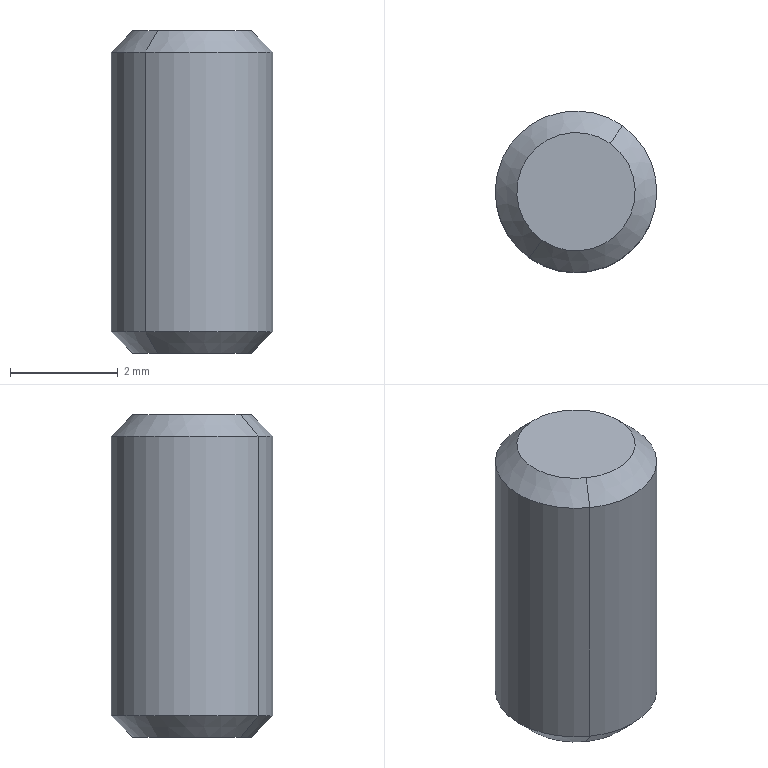Component | SolidWorks | Part28-2 | 1 solid | 8 faces | box 3 x 3 x 6 mm | volume 41 mm3 | cone 4 | cylinder 2 | plane 2 | commonest cylinder face diameters 3 x2
build123d program:
from build123d import *

# Parameters (mm, degrees)
SKETCH1_R           = 1.5
BOSS_EXTRUDE1_DEPTH = 6
CHAMFER1_SIZE       = 0.4


with BuildPart() as part:
    # Sketch1 → Boss-Extrude1 (new body)
    with BuildSketch(Plane.XY):
        Circle(SKETCH1_R)
    extrude(amount=BOSS_EXTRUDE1_DEPTH)

    # Chamfer1
    chamfer1_edges = [part.edges().sort_by_distance(p)[0] for p in [
        (-1.5, 0, 0),
        (-1.5, 0, 6),
    ]]
    chamfer(chamfer1_edges, length=CHAMFER1_SIZE)


solid = part.part

# Placed as in the assembly
solid = solid.moved(Location((65.747, 35.686, -29.938), (0, 0, 0)))
STEP:
#1=COLOUR_RGB('',0.7922,0.8196,0.9333);
#2=FILL_AREA_STYLE_COLOUR('',#1);
#3=FILL_AREA_STYLE('',(#2));
#4=SURFACE_STYLE_FILL_AREA(#3);
#5=SURFACE_SIDE_STYLE('',(#4));
#6=SURFACE_STYLE_USAGE(.BOTH.,#5);
#7=PRESENTATION_STYLE_ASSIGNMENT((#6));
#8=CARTESIAN_POINT('',(2.564,1.37,-0.9424));
#9=VERTEX_POINT('',#8);
#10=CARTESIAN_POINT('',(2.613,1.44,-0.9424));
#11=VERTEX_POINT('',#10);
#12=CARTESIAN_POINT('',(2.588,1.405,-0.9424));
#13=DIRECTION('',(0.,-0.,1.));
#14=DIRECTION('',(-0.5758,-0.8176,0.));
#15=AXIS2_PLACEMENT_3D('',#12,#13,#14);
#16=CIRCLE('',#15,0.04331);
#17=EDGE_CURVE('',#9,#11,#16,.T.);
#18=ORIENTED_EDGE('',*,*,#17,.F.);
#19=CARTESIAN_POINT('',(2.554,1.357,-0.9582));
#20=VERTEX_POINT('',#19);
#21=CARTESIAN_POINT('',(2.564,1.37,-0.9424));
#22=DIRECTION('',(-0.4072,-0.5781,-0.7071));
#23=VECTOR('',#22,39.37);
#24=LINE('',#21,#23);
#25=EDGE_CURVE('',#9,#20,#24,.T.);
#26=ORIENTED_EDGE('',*,*,#25,.T.);
#27=CARTESIAN_POINT('',(2.622,1.453,-0.9582));
#28=VERTEX_POINT('',#27);
#29=CARTESIAN_POINT('',(2.588,1.405,-0.9582));
#30=DIRECTION('',(-0.,0.,-1.));
#31=DIRECTION('',(-0.5758,-0.8176,0.));
#32=AXIS2_PLACEMENT_3D('',#29,#30,#31);
#33=CIRCLE('',#32,0.05906);
#34=EDGE_CURVE('',#28,#20,#33,.T.);
#35=ORIENTED_EDGE('',*,*,#34,.F.);
#36=CARTESIAN_POINT('',(2.613,1.44,-0.9424));
#37=DIRECTION('',(0.4072,0.5781,-0.7071));
#38=VECTOR('',#37,39.37);
#39=LINE('',#36,#38);
#40=EDGE_CURVE('',#11,#28,#39,.T.);
#41=ORIENTED_EDGE('',*,*,#40,.F.);
#42=EDGE_LOOP('',(#18,#26,#35,#41));
#43=FACE_OUTER_BOUND('',#42,.T.);
#44=CARTESIAN_POINT('',(2.588,1.405,-0.9424));
#45=DIRECTION('',(-0.,0.,-1.));
#46=DIRECTION('',(0.5758,0.8176,0.));
#47=AXIS2_PLACEMENT_3D('',#44,#45,#46);
#48=CONICAL_SURFACE('',#47,0.04331,0.7854);
#49=ADVANCED_FACE('',(#43),#48,.T.);
#50=CARTESIAN_POINT('',(2.613,1.44,-1.179));
#51=VERTEX_POINT('',#50);
#52=CARTESIAN_POINT('',(2.564,1.37,-1.179));
#53=VERTEX_POINT('',#52);
#54=CARTESIAN_POINT('',(2.588,1.405,-1.179));
#55=DIRECTION('',(-0.,0.,-1.));
#56=DIRECTION('',(-0.5758,-0.8176,0.));
#57=AXIS2_PLACEMENT_3D('',#54,#55,#56);
#58=CIRCLE('',#57,0.04331);
#59=EDGE_CURVE('',#51,#53,#58,.T.);
#60=ORIENTED_EDGE('',*,*,#59,.F.);
#61=CARTESIAN_POINT('',(2.622,1.453,-1.163));
#62=VERTEX_POINT('',#61);
#63=CARTESIAN_POINT('',(2.622,1.453,-1.163));
#64=DIRECTION('',(0.4072,0.5781,0.7071));
#65=VECTOR('',#64,39.37);
#66=LINE('',#63,#65);
#67=EDGE_CURVE('',#51,#62,#66,.T.);
#68=ORIENTED_EDGE('',*,*,#67,.T.);
#69=CARTESIAN_POINT('',(2.554,1.357,-1.163));
#70=VERTEX_POINT('',#69);
#71=CARTESIAN_POINT('',(2.588,1.405,-1.163));
#72=DIRECTION('',(0.,-0.,1.));
#73=DIRECTION('',(-0.5758,-0.8176,0.));
#74=AXIS2_PLACEMENT_3D('',#71,#72,#73);
#75=CIRCLE('',#74,0.05906);
#76=EDGE_CURVE('',#70,#62,#75,.T.);
#77=ORIENTED_EDGE('',*,*,#76,.F.);
#78=CARTESIAN_POINT('',(2.554,1.357,-1.163));
#79=DIRECTION('',(-0.4072,-0.5781,0.7071));
#80=VECTOR('',#79,39.37);
#81=LINE('',#78,#80);
#82=EDGE_CURVE('',#53,#70,#81,.T.);
#83=ORIENTED_EDGE('',*,*,#82,.F.);
#84=EDGE_LOOP('',(#60,#68,#77,#83));
#85=FACE_OUTER_BOUND('',#84,.T.);
#86=CARTESIAN_POINT('',(2.588,1.405,-1.163));
#87=DIRECTION('',(0.,-0.,1.));
#88=DIRECTION('',(-0.5758,-0.8176,0.));
#89=AXIS2_PLACEMENT_3D('',#86,#87,#88);
#90=CONICAL_SURFACE('',#89,0.05906,0.7854);
#91=ADVANCED_FACE('',(#85),#90,.T.);
#92=ORIENTED_EDGE('',*,*,#34,.T.);
#93=CARTESIAN_POINT('',(2.554,1.357,-0.9424));
#94=DIRECTION('',(-0.,0.,-1.));
#95=VECTOR('',#94,39.37);
#96=LINE('',#93,#95);
#97=EDGE_CURVE('',#20,#70,#96,.T.);
#98=ORIENTED_EDGE('',*,*,#97,.T.);
#99=ORIENTED_EDGE('',*,*,#76,.T.);
#100=CARTESIAN_POINT('',(2.622,1.453,-0.9424));
#101=DIRECTION('',(-0.,0.,-1.));
#102=VECTOR('',#101,39.37);
#103=LINE('',#100,#102);
#104=EDGE_CURVE('',#28,#62,#103,.T.);
#105=ORIENTED_EDGE('',*,*,#104,.F.);
#106=EDGE_LOOP('',(#92,#98,#99,#105));
#107=FACE_OUTER_BOUND('',#106,.T.);
#108=CARTESIAN_POINT('',(2.588,1.405,-0.9424));
#109=DIRECTION('',(-0.,0.,-1.));
#110=DIRECTION('',(0.5758,0.8176,0.));
#111=AXIS2_PLACEMENT_3D('',#108,#109,#110);
#112=CYLINDRICAL_SURFACE('',#111,0.05906);
#113=ADVANCED_FACE('',(#107),#112,.T.);
#114=ORIENTED_EDGE('',*,*,#97,.F.);
#115=CARTESIAN_POINT('',(2.588,1.405,-0.9582));
#116=DIRECTION('',(-0.,0.,-1.));
#117=DIRECTION('',(-0.5758,-0.8176,0.));
#118=AXIS2_PLACEMENT_3D('',#115,#116,#117);
#119=CIRCLE('',#118,0.05906);
#120=EDGE_CURVE('',#20,#28,#119,.T.);
#121=ORIENTED_EDGE('',*,*,#120,.T.);
#122=ORIENTED_EDGE('',*,*,#104,.T.);
#123=CARTESIAN_POINT('',(2.588,1.405,-1.163));
#124=DIRECTION('',(0.,-0.,1.));
#125=DIRECTION('',(-0.5758,-0.8176,0.));
#126=AXIS2_PLACEMENT_3D('',#123,#124,#125);
#127=CIRCLE('',#126,0.05906);
#128=EDGE_CURVE('',#62,#70,#127,.T.);
#129=ORIENTED_EDGE('',*,*,#128,.T.);
#130=EDGE_LOOP('',(#114,#121,#122,#129));
#131=FACE_OUTER_BOUND('',#130,.T.);
#132=CARTESIAN_POINT('',(2.588,1.405,-0.9424));
#133=DIRECTION('',(-0.,0.,-1.));
#134=DIRECTION('',(0.5758,0.8176,0.));
#135=AXIS2_PLACEMENT_3D('',#132,#133,#134);
#136=CYLINDRICAL_SURFACE('',#135,0.05906);
#137=ADVANCED_FACE('',(#131),#136,.T.);
#138=CARTESIAN_POINT('',(2.588,1.405,-0.9424));
#139=DIRECTION('',(0.,-0.,1.));
#140=DIRECTION('',(-0.5758,-0.8176,0.));
#141=AXIS2_PLACEMENT_3D('',#138,#139,#140);
#142=CIRCLE('',#141,0.04331);
#143=EDGE_CURVE('',#11,#9,#142,.T.);
#144=ORIENTED_EDGE('',*,*,#143,.T.);
#145=ORIENTED_EDGE('',*,*,#17,.T.);
#146=EDGE_LOOP('',(#144,#145));
#147=FACE_OUTER_BOUND('',#146,.T.);
#148=CARTESIAN_POINT('',(2.588,1.405,-0.9424));
#149=DIRECTION('',(0.,-0.,1.));
#150=DIRECTION('',(-0.5758,-0.8176,0.));
#151=AXIS2_PLACEMENT_3D('',#148,#149,#150);
#152=PLANE('',#151);
#153=ADVANCED_FACE('',(#147),#152,.T.);
#154=CARTESIAN_POINT('',(2.588,1.405,-1.179));
#155=DIRECTION('',(-0.,0.,-1.));
#156=DIRECTION('',(-0.5758,-0.8176,0.));
#157=AXIS2_PLACEMENT_3D('',#154,#155,#156);
#158=CIRCLE('',#157,0.04331);
#159=EDGE_CURVE('',#53,#51,#158,.T.);
#160=ORIENTED_EDGE('',*,*,#159,.T.);
#161=ORIENTED_EDGE('',*,*,#59,.T.);
#162=EDGE_LOOP('',(#160,#161));
#163=FACE_OUTER_BOUND('',#162,.T.);
#164=CARTESIAN_POINT('',(2.588,1.405,-1.179));
#165=DIRECTION('',(0.,-0.,1.));
#166=DIRECTION('',(-0.5758,-0.8176,0.));
#167=AXIS2_PLACEMENT_3D('',#164,#165,#166);
#168=PLANE('',#167);
#169=ADVANCED_FACE('',(#163),#168,.F.);
#170=ORIENTED_EDGE('',*,*,#67,.F.);
#171=ORIENTED_EDGE('',*,*,#159,.F.);
#172=ORIENTED_EDGE('',*,*,#82,.T.);
#173=ORIENTED_EDGE('',*,*,#128,.F.);
#174=EDGE_LOOP('',(#170,#171,#172,#173));
#175=FACE_OUTER_BOUND('',#174,.T.);
#176=CARTESIAN_POINT('',(2.588,1.405,-1.163));
#177=DIRECTION('',(0.,-0.,1.));
#178=DIRECTION('',(-0.5758,-0.8176,0.));
#179=AXIS2_PLACEMENT_3D('',#176,#177,#178);
#180=CONICAL_SURFACE('',#179,0.05906,0.7854);
#181=ADVANCED_FACE('',(#175),#180,.T.);
#182=ORIENTED_EDGE('',*,*,#25,.F.);
#183=ORIENTED_EDGE('',*,*,#143,.F.);
#184=ORIENTED_EDGE('',*,*,#40,.T.);
#185=ORIENTED_EDGE('',*,*,#120,.F.);
#186=EDGE_LOOP('',(#182,#183,#184,#185));
#187=FACE_OUTER_BOUND('',#186,.T.);
#188=CARTESIAN_POINT('',(2.588,1.405,-0.9424));
#189=DIRECTION('',(-0.,0.,-1.));
#190=DIRECTION('',(0.5758,0.8176,0.));
#191=AXIS2_PLACEMENT_3D('',#188,#189,#190);
#192=CONICAL_SURFACE('',#191,0.04331,0.7854);
#193=ADVANCED_FACE('',(#187),#192,.T.);
#194=CLOSED_SHELL('',(#49,#91,#113,#137,#153,#169,#181,#193));
#195=MANIFOLD_SOLID_BREP('',#194);
#196=STYLED_ITEM('',(#7),#195);
#197=(LENGTH_UNIT()NAMED_UNIT(*)SI_UNIT($,.METRE.));
#198=LENGTH_MEASURE_WITH_UNIT(LENGTH_MEASURE(0.0254),#197);
#199=DIMENSIONAL_EXPONENTS(1.,0.,0.,0.,0.,0.,0.);
#200=(CONVERSION_BASED_UNIT('',#198)LENGTH_UNIT()NAMED_UNIT(#199));
#201=UNCERTAINTY_MEASURE_WITH_UNIT(LENGTH_MEASURE(0.00001),#200,'','');
#202=(NAMED_UNIT(*)PLANE_ANGLE_UNIT()SI_UNIT($,.RADIAN.));
#203=(NAMED_UNIT(*)SI_UNIT($,.STERADIAN.)SOLID_ANGLE_UNIT());
#204=(GEOMETRIC_REPRESENTATION_CONTEXT(3)GLOBAL_UNCERTAINTY_ASSIGNED_CONTEXT((#201))GLOBAL_UNIT_ASSIGNED_CONTEXT((#200,#202,#203))REPRESENTATION_CONTEXT('',''));
#205=MECHANICAL_DESIGN_GEOMETRIC_PRESENTATION_REPRESENTATION('',(#196),#204);
#206=CARTESIAN_POINT('',(0.,0.,0.));
#207=DIRECTION('',(0.,0.,1.));
#208=DIRECTION('',(1.,0.,0.));
#209=AXIS2_PLACEMENT_3D('',#206,#207,#208);
#210=(LENGTH_UNIT()NAMED_UNIT(*)SI_UNIT($,.METRE.));
#211=LENGTH_MEASURE_WITH_UNIT(LENGTH_MEASURE(0.0254),#210);
#212=DIMENSIONAL_EXPONENTS(1.,0.,0.,0.,0.,0.,0.);
#213=(CONVERSION_BASED_UNIT('',#211)LENGTH_UNIT()NAMED_UNIT(#212));
#214=UNCERTAINTY_MEASURE_WITH_UNIT(LENGTH_MEASURE(0.00001),#213,'','');
#215=(NAMED_UNIT(*)PLANE_ANGLE_UNIT()SI_UNIT($,.RADIAN.));
#216=(NAMED_UNIT(*)SI_UNIT($,.STERADIAN.)SOLID_ANGLE_UNIT());
#217=(GEOMETRIC_REPRESENTATION_CONTEXT(3)GLOBAL_UNCERTAINTY_ASSIGNED_CONTEXT((#214))GLOBAL_UNIT_ASSIGNED_CONTEXT((#213,#215,#216))REPRESENTATION_CONTEXT('',''));
#218=ADVANCED_BREP_SHAPE_REPRESENTATION('',(#195,#209),#217);
#219=PRESENTATION_LAYER_ASSIGNMENT('','',(#196));